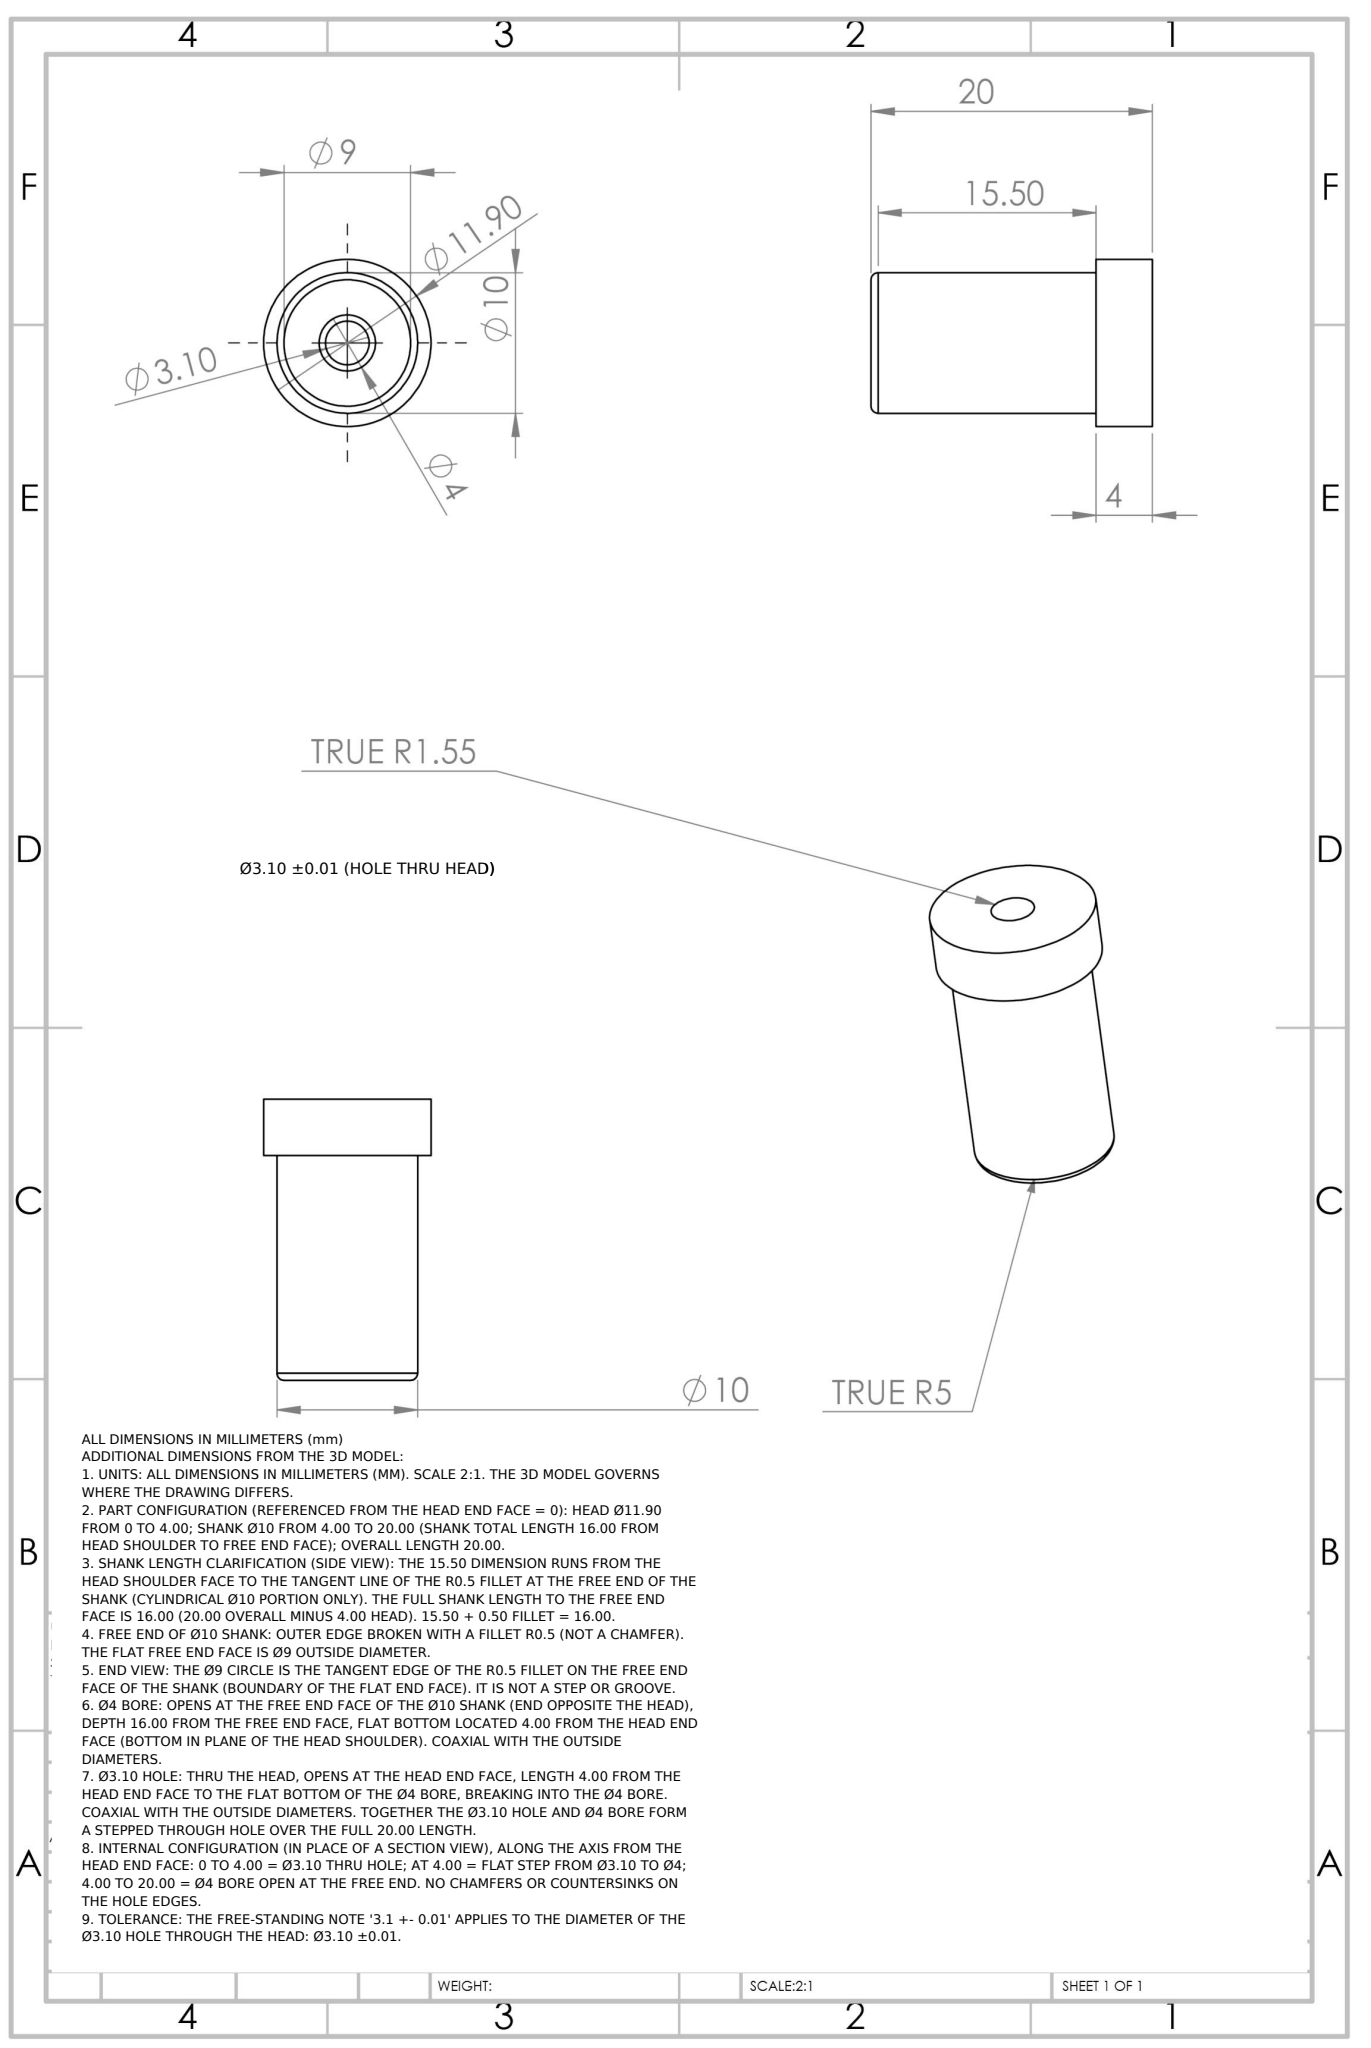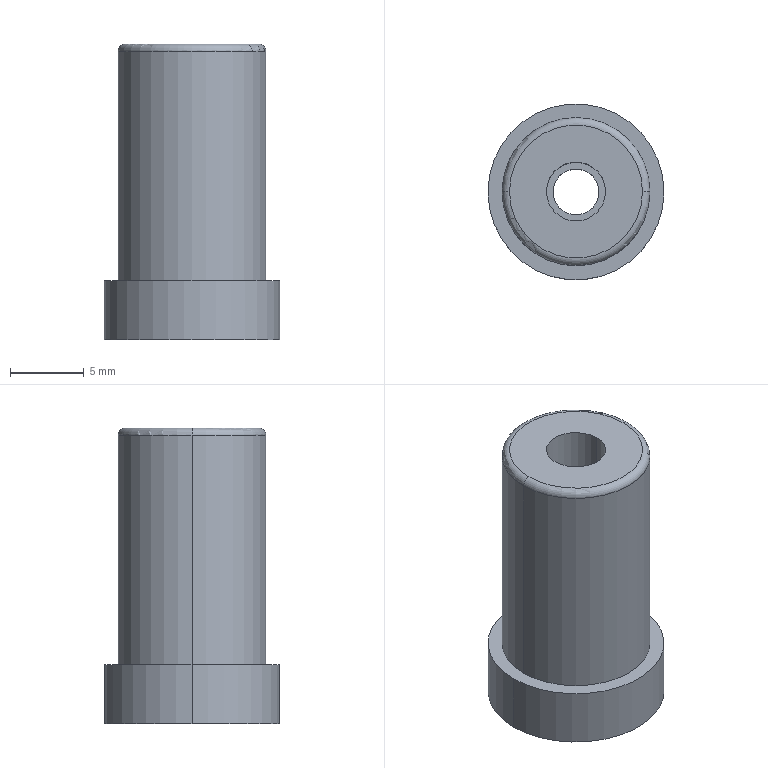Part | NX | mm | Flanged Cylindrical Bore Bushing | 1 solid | 14 faces | box 11.9 x 11.9 x 20 mm | volume 1469 mm3 | cylinder 8 | plane 4 | torus 2 | commonest cylinder face diameters 4 x2 10 x2 11.9 x2 3.1 x2
STEP:
#1=COLOUR_RGB('',1.,0.7529,1.);
#2=FILL_AREA_STYLE_COLOUR('',#1);
#3=FILL_AREA_STYLE('',(#2));
#4=SURFACE_STYLE_FILL_AREA(#3);
#5=SURFACE_SIDE_STYLE('',(#4));
#6=SURFACE_STYLE_USAGE(.BOTH.,#5);
#7=PRESENTATION_STYLE_ASSIGNMENT((#6));
#8=CARTESIAN_POINT('',(-2.,0.,4.));
#9=VERTEX_POINT('',#8);
#10=CARTESIAN_POINT('',(2.,0.,4.));
#11=VERTEX_POINT('',#10);
#12=CARTESIAN_POINT('',(0.,0.,4.));
#13=DIRECTION('',(0.,0.,1.));
#14=DIRECTION('',(1.,0.,0.));
#15=AXIS2_PLACEMENT_3D('',#12,#13,#14);
#16=CIRCLE('',#15,2.);
#17=EDGE_CURVE('',#9,#11,#16,.T.);
#18=ORIENTED_EDGE('',*,*,#17,.F.);
#19=CARTESIAN_POINT('',(-2.,0.,20.));
#20=VERTEX_POINT('',#19);
#21=CARTESIAN_POINT('',(-2.,0.,4.));
#22=DIRECTION('',(0.,0.,1.));
#23=VECTOR('',#22,1000.);
#24=LINE('',#21,#23);
#25=EDGE_CURVE('',#9,#20,#24,.T.);
#26=ORIENTED_EDGE('',*,*,#25,.T.);
#27=CARTESIAN_POINT('',(2.,0.,20.));
#28=VERTEX_POINT('',#27);
#29=CARTESIAN_POINT('',(0.,0.,20.));
#30=DIRECTION('',(0.,0.,1.));
#31=DIRECTION('',(1.,0.,0.));
#32=AXIS2_PLACEMENT_3D('',#29,#30,#31);
#33=CIRCLE('',#32,2.);
#34=EDGE_CURVE('',#20,#28,#33,.T.);
#35=ORIENTED_EDGE('',*,*,#34,.T.);
#36=CARTESIAN_POINT('',(2.,0.,4.));
#37=DIRECTION('',(0.,0.,1.));
#38=VECTOR('',#37,1000.);
#39=LINE('',#36,#38);
#40=EDGE_CURVE('',#11,#28,#39,.T.);
#41=ORIENTED_EDGE('',*,*,#40,.F.);
#42=EDGE_LOOP('',(#18,#26,#35,#41));
#43=FACE_OUTER_BOUND('',#42,.T.);
#44=CARTESIAN_POINT('',(0.,0.,4.));
#45=DIRECTION('',(0.,0.,1.));
#46=DIRECTION('',(1.,0.,0.));
#47=AXIS2_PLACEMENT_3D('',#44,#45,#46);
#48=CYLINDRICAL_SURFACE('',#47,2.);
#49=ADVANCED_FACE('',(#43),#48,.F.);
#50=CARTESIAN_POINT('',(-5.,0.,19.5));
#51=VERTEX_POINT('',#50);
#52=CARTESIAN_POINT('',(5.,0.,19.5));
#53=VERTEX_POINT('',#52);
#54=CARTESIAN_POINT('',(0.,0.,19.5));
#55=DIRECTION('',(0.,0.,-1.));
#56=DIRECTION('',(1.,0.,0.));
#57=AXIS2_PLACEMENT_3D('',#54,#55,#56);
#58=CIRCLE('',#57,5.);
#59=EDGE_CURVE('',#51,#53,#58,.T.);
#60=ORIENTED_EDGE('',*,*,#59,.F.);
#61=CARTESIAN_POINT('',(-4.5,0.,20.));
#62=VERTEX_POINT('',#61);
#63=CARTESIAN_POINT('',(-4.5,0.,19.5));
#64=DIRECTION('',(0.,1.,0.));
#65=DIRECTION('',(-1.,0.,0.));
#66=AXIS2_PLACEMENT_3D('',#63,#64,#65);
#67=CIRCLE('',#66,0.5);
#68=EDGE_CURVE('',#51,#62,#67,.T.);
#69=ORIENTED_EDGE('',*,*,#68,.T.);
#70=CARTESIAN_POINT('',(4.5,0.,20.));
#71=VERTEX_POINT('',#70);
#72=CARTESIAN_POINT('',(0.,0.,20.));
#73=DIRECTION('',(0.,0.,1.));
#74=DIRECTION('',(1.,0.,0.));
#75=AXIS2_PLACEMENT_3D('',#72,#73,#74);
#76=CIRCLE('',#75,4.5);
#77=EDGE_CURVE('',#71,#62,#76,.T.);
#78=ORIENTED_EDGE('',*,*,#77,.F.);
#79=CARTESIAN_POINT('',(4.5,0.,19.5));
#80=DIRECTION('',(0.,-1.,0.));
#81=DIRECTION('',(0.,0.,-1.));
#82=AXIS2_PLACEMENT_3D('',#79,#80,#81);
#83=CIRCLE('',#82,0.5);
#84=EDGE_CURVE('',#53,#71,#83,.T.);
#85=ORIENTED_EDGE('',*,*,#84,.F.);
#86=EDGE_LOOP('',(#60,#69,#78,#85));
#87=FACE_OUTER_BOUND('',#86,.T.);
#88=CARTESIAN_POINT('',(0.,0.,19.5));
#89=DIRECTION('',(0.,0.,1.));
#90=DIRECTION('',(1.,0.,0.));
#91=AXIS2_PLACEMENT_3D('',#88,#89,#90);
#92=TOROIDAL_SURFACE('',#91,4.5,0.5);
#93=ADVANCED_FACE('',(#87),#92,.T.);
#94=CARTESIAN_POINT('',(5.,0.,4.));
#95=VERTEX_POINT('',#94);
#96=CARTESIAN_POINT('',(-5.,0.,4.));
#97=VERTEX_POINT('',#96);
#98=CARTESIAN_POINT('',(0.,0.,4.));
#99=DIRECTION('',(0.,0.,1.));
#100=DIRECTION('',(1.,0.,0.));
#101=AXIS2_PLACEMENT_3D('',#98,#99,#100);
#102=CIRCLE('',#101,5.);
#103=EDGE_CURVE('',#95,#97,#102,.T.);
#104=ORIENTED_EDGE('',*,*,#103,.T.);
#105=CARTESIAN_POINT('',(-5.,0.,4.));
#106=DIRECTION('',(0.,0.,1.));
#107=VECTOR('',#106,1000.);
#108=LINE('',#105,#107);
#109=EDGE_CURVE('',#97,#51,#108,.T.);
#110=ORIENTED_EDGE('',*,*,#109,.T.);
#111=ORIENTED_EDGE('',*,*,#59,.T.);
#112=CARTESIAN_POINT('',(5.,0.,4.));
#113=DIRECTION('',(0.,0.,1.));
#114=VECTOR('',#113,1000.);
#115=LINE('',#112,#114);
#116=EDGE_CURVE('',#95,#53,#115,.T.);
#117=ORIENTED_EDGE('',*,*,#116,.F.);
#118=EDGE_LOOP('',(#104,#110,#111,#117));
#119=FACE_OUTER_BOUND('',#118,.T.);
#120=CARTESIAN_POINT('',(0.,0.,4.));
#121=DIRECTION('',(0.,0.,1.));
#122=DIRECTION('',(1.,0.,0.));
#123=AXIS2_PLACEMENT_3D('',#120,#121,#122);
#124=CYLINDRICAL_SURFACE('',#123,5.);
#125=ADVANCED_FACE('',(#119),#124,.T.);
#126=CARTESIAN_POINT('',(5.95,0.,4.));
#127=VERTEX_POINT('',#126);
#128=CARTESIAN_POINT('',(-5.95,0.,4.));
#129=VERTEX_POINT('',#128);
#130=CARTESIAN_POINT('',(0.,0.,4.));
#131=DIRECTION('',(0.,0.,1.));
#132=DIRECTION('',(1.,0.,0.));
#133=AXIS2_PLACEMENT_3D('',#130,#131,#132);
#134=CIRCLE('',#133,5.95);
#135=EDGE_CURVE('',#127,#129,#134,.T.);
#136=ORIENTED_EDGE('',*,*,#135,.F.);
#137=CARTESIAN_POINT('',(5.95,0.,0.));
#138=VERTEX_POINT('',#137);
#139=CARTESIAN_POINT('',(5.95,0.,20.));
#140=DIRECTION('',(0.,0.,-1.));
#141=VECTOR('',#140,1000.);
#142=LINE('',#139,#141);
#143=EDGE_CURVE('',#127,#138,#142,.T.);
#144=ORIENTED_EDGE('',*,*,#143,.T.);
#145=CARTESIAN_POINT('',(-5.95,0.,0.));
#146=VERTEX_POINT('',#145);
#147=CARTESIAN_POINT('',(0.,0.,0.));
#148=DIRECTION('',(0.,0.,1.));
#149=DIRECTION('',(1.,0.,0.));
#150=AXIS2_PLACEMENT_3D('',#147,#148,#149);
#151=CIRCLE('',#150,5.95);
#152=EDGE_CURVE('',#138,#146,#151,.T.);
#153=ORIENTED_EDGE('',*,*,#152,.T.);
#154=CARTESIAN_POINT('',(-5.95,0.,20.));
#155=DIRECTION('',(0.,0.,-1.));
#156=VECTOR('',#155,1000.);
#157=LINE('',#154,#156);
#158=EDGE_CURVE('',#129,#146,#157,.T.);
#159=ORIENTED_EDGE('',*,*,#158,.F.);
#160=EDGE_LOOP('',(#136,#144,#153,#159));
#161=FACE_OUTER_BOUND('',#160,.T.);
#162=CARTESIAN_POINT('',(0.,0.,20.));
#163=DIRECTION('',(0.,0.,-1.));
#164=DIRECTION('',(-1.,0.,0.));
#165=AXIS2_PLACEMENT_3D('',#162,#163,#164);
#166=CYLINDRICAL_SURFACE('',#165,5.95);
#167=ADVANCED_FACE('',(#161),#166,.T.);
#168=CARTESIAN_POINT('',(1.55,0.,4.));
#169=VERTEX_POINT('',#168);
#170=CARTESIAN_POINT('',(-1.55,0.,4.));
#171=VERTEX_POINT('',#170);
#172=CARTESIAN_POINT('',(0.,0.,4.));
#173=DIRECTION('',(0.,0.,-1.));
#174=DIRECTION('',(1.,0.,0.));
#175=AXIS2_PLACEMENT_3D('',#172,#173,#174);
#176=CIRCLE('',#175,1.55);
#177=EDGE_CURVE('',#169,#171,#176,.T.);
#178=ORIENTED_EDGE('',*,*,#177,.F.);
#179=CARTESIAN_POINT('',(1.55,0.,0.));
#180=VERTEX_POINT('',#179);
#181=CARTESIAN_POINT('',(1.55,0.,20.));
#182=DIRECTION('',(0.,0.,-1.));
#183=VECTOR('',#182,1000.);
#184=LINE('',#181,#183);
#185=EDGE_CURVE('',#169,#180,#184,.T.);
#186=ORIENTED_EDGE('',*,*,#185,.T.);
#187=CARTESIAN_POINT('',(-1.55,0.,0.));
#188=VERTEX_POINT('',#187);
#189=CARTESIAN_POINT('',(0.,0.,0.));
#190=DIRECTION('',(0.,0.,-1.));
#191=DIRECTION('',(-1.,0.,0.));
#192=AXIS2_PLACEMENT_3D('',#189,#190,#191);
#193=CIRCLE('',#192,1.55);
#194=EDGE_CURVE('',#180,#188,#193,.T.);
#195=ORIENTED_EDGE('',*,*,#194,.T.);
#196=CARTESIAN_POINT('',(-1.55,0.,20.));
#197=DIRECTION('',(0.,0.,-1.));
#198=VECTOR('',#197,1000.);
#199=LINE('',#196,#198);
#200=EDGE_CURVE('',#171,#188,#199,.T.);
#201=ORIENTED_EDGE('',*,*,#200,.F.);
#202=EDGE_LOOP('',(#178,#186,#195,#201));
#203=FACE_OUTER_BOUND('',#202,.T.);
#204=CARTESIAN_POINT('',(0.,0.,20.));
#205=DIRECTION('',(0.,0.,-1.));
#206=DIRECTION('',(-1.,0.,0.));
#207=AXIS2_PLACEMENT_3D('',#204,#205,#206);
#208=CYLINDRICAL_SURFACE('',#207,1.55);
#209=ADVANCED_FACE('',(#203),#208,.F.);
#210=ORIENTED_EDGE('',*,*,#185,.F.);
#211=CARTESIAN_POINT('',(0.,0.,4.));
#212=DIRECTION('',(0.,0.,-1.));
#213=DIRECTION('',(1.,0.,0.));
#214=AXIS2_PLACEMENT_3D('',#211,#212,#213);
#215=CIRCLE('',#214,1.55);
#216=EDGE_CURVE('',#171,#169,#215,.T.);
#217=ORIENTED_EDGE('',*,*,#216,.F.);
#218=ORIENTED_EDGE('',*,*,#200,.T.);
#219=CARTESIAN_POINT('',(0.,0.,0.));
#220=DIRECTION('',(0.,0.,-1.));
#221=DIRECTION('',(-1.,0.,0.));
#222=AXIS2_PLACEMENT_3D('',#219,#220,#221);
#223=CIRCLE('',#222,1.55);
#224=EDGE_CURVE('',#188,#180,#223,.T.);
#225=ORIENTED_EDGE('',*,*,#224,.T.);
#226=EDGE_LOOP('',(#210,#217,#218,#225));
#227=FACE_OUTER_BOUND('',#226,.T.);
#228=CARTESIAN_POINT('',(0.,0.,20.));
#229=DIRECTION('',(0.,0.,-1.));
#230=DIRECTION('',(-1.,0.,0.));
#231=AXIS2_PLACEMENT_3D('',#228,#229,#230);
#232=CYLINDRICAL_SURFACE('',#231,1.55);
#233=ADVANCED_FACE('',(#227),#232,.F.);
#234=ORIENTED_EDGE('',*,*,#143,.F.);
#235=CARTESIAN_POINT('',(0.,0.,4.));
#236=DIRECTION('',(0.,0.,1.));
#237=DIRECTION('',(1.,0.,0.));
#238=AXIS2_PLACEMENT_3D('',#235,#236,#237);
#239=CIRCLE('',#238,5.95);
#240=EDGE_CURVE('',#129,#127,#239,.T.);
#241=ORIENTED_EDGE('',*,*,#240,.F.);
#242=ORIENTED_EDGE('',*,*,#158,.T.);
#243=CARTESIAN_POINT('',(0.,0.,0.));
#244=DIRECTION('',(0.,0.,1.));
#245=DIRECTION('',(1.,0.,0.));
#246=AXIS2_PLACEMENT_3D('',#243,#244,#245);
#247=CIRCLE('',#246,5.95);
#248=EDGE_CURVE('',#146,#138,#247,.T.);
#249=ORIENTED_EDGE('',*,*,#248,.T.);
#250=EDGE_LOOP('',(#234,#241,#242,#249));
#251=FACE_OUTER_BOUND('',#250,.T.);
#252=CARTESIAN_POINT('',(0.,0.,20.));
#253=DIRECTION('',(0.,0.,-1.));
#254=DIRECTION('',(-1.,0.,0.));
#255=AXIS2_PLACEMENT_3D('',#252,#253,#254);
#256=CYLINDRICAL_SURFACE('',#255,5.95);
#257=ADVANCED_FACE('',(#251),#256,.T.);
#258=ORIENTED_EDGE('',*,*,#224,.F.);
#259=ORIENTED_EDGE('',*,*,#194,.F.);
#260=EDGE_LOOP('',(#258,#259));
#261=FACE_BOUND('',#260,.T.);
#262=ORIENTED_EDGE('',*,*,#248,.F.);
#263=ORIENTED_EDGE('',*,*,#152,.F.);
#264=EDGE_LOOP('',(#262,#263));
#265=FACE_OUTER_BOUND('',#264,.T.);
#266=CARTESIAN_POINT('',(0.,0.,0.));
#267=DIRECTION('',(0.,0.,1.));
#268=DIRECTION('',(1.,0.,0.));
#269=AXIS2_PLACEMENT_3D('',#266,#267,#268);
#270=PLANE('',#269);
#271=ADVANCED_FACE('',(#261,#265),#270,.F.);
#272=ORIENTED_EDGE('',*,*,#103,.F.);
#273=CARTESIAN_POINT('',(0.,0.,4.));
#274=DIRECTION('',(0.,0.,1.));
#275=DIRECTION('',(1.,0.,0.));
#276=AXIS2_PLACEMENT_3D('',#273,#274,#275);
#277=CIRCLE('',#276,5.);
#278=EDGE_CURVE('',#97,#95,#277,.T.);
#279=ORIENTED_EDGE('',*,*,#278,.F.);
#280=EDGE_LOOP('',(#272,#279));
#281=FACE_BOUND('',#280,.T.);
#282=ORIENTED_EDGE('',*,*,#240,.T.);
#283=ORIENTED_EDGE('',*,*,#135,.T.);
#284=EDGE_LOOP('',(#282,#283));
#285=FACE_OUTER_BOUND('',#284,.T.);
#286=CARTESIAN_POINT('',(0.,0.,4.));
#287=DIRECTION('',(0.,0.,1.));
#288=DIRECTION('',(1.,0.,0.));
#289=AXIS2_PLACEMENT_3D('',#286,#287,#288);
#290=PLANE('',#289);
#291=ADVANCED_FACE('',(#281,#285),#290,.T.);
#292=ORIENTED_EDGE('',*,*,#109,.F.);
#293=ORIENTED_EDGE('',*,*,#278,.T.);
#294=ORIENTED_EDGE('',*,*,#116,.T.);
#295=CARTESIAN_POINT('',(0.,0.,19.5));
#296=DIRECTION('',(0.,0.,-1.));
#297=DIRECTION('',(1.,0.,0.));
#298=AXIS2_PLACEMENT_3D('',#295,#296,#297);
#299=CIRCLE('',#298,5.);
#300=EDGE_CURVE('',#53,#51,#299,.T.);
#301=ORIENTED_EDGE('',*,*,#300,.T.);
#302=EDGE_LOOP('',(#292,#293,#294,#301));
#303=FACE_OUTER_BOUND('',#302,.T.);
#304=CARTESIAN_POINT('',(0.,0.,4.));
#305=DIRECTION('',(0.,0.,1.));
#306=DIRECTION('',(1.,0.,0.));
#307=AXIS2_PLACEMENT_3D('',#304,#305,#306);
#308=CYLINDRICAL_SURFACE('',#307,5.);
#309=ADVANCED_FACE('',(#303),#308,.T.);
#310=CARTESIAN_POINT('',(0.,0.,20.));
#311=DIRECTION('',(0.,0.,1.));
#312=DIRECTION('',(1.,0.,0.));
#313=AXIS2_PLACEMENT_3D('',#310,#311,#312);
#314=CIRCLE('',#313,2.);
#315=EDGE_CURVE('',#28,#20,#314,.T.);
#316=ORIENTED_EDGE('',*,*,#315,.F.);
#317=ORIENTED_EDGE('',*,*,#34,.F.);
#318=EDGE_LOOP('',(#316,#317));
#319=FACE_BOUND('',#318,.T.);
#320=ORIENTED_EDGE('',*,*,#77,.T.);
#321=CARTESIAN_POINT('',(0.,0.,20.));
#322=DIRECTION('',(0.,0.,1.));
#323=DIRECTION('',(1.,0.,0.));
#324=AXIS2_PLACEMENT_3D('',#321,#322,#323);
#325=CIRCLE('',#324,4.5);
#326=EDGE_CURVE('',#62,#71,#325,.T.);
#327=ORIENTED_EDGE('',*,*,#326,.T.);
#328=EDGE_LOOP('',(#320,#327));
#329=FACE_OUTER_BOUND('',#328,.T.);
#330=CARTESIAN_POINT('',(0.,0.,20.));
#331=DIRECTION('',(0.,0.,1.));
#332=DIRECTION('',(1.,0.,0.));
#333=AXIS2_PLACEMENT_3D('',#330,#331,#332);
#334=PLANE('',#333);
#335=ADVANCED_FACE('',(#319,#329),#334,.T.);
#336=ORIENTED_EDGE('',*,*,#68,.F.);
#337=ORIENTED_EDGE('',*,*,#300,.F.);
#338=ORIENTED_EDGE('',*,*,#84,.T.);
#339=ORIENTED_EDGE('',*,*,#326,.F.);
#340=EDGE_LOOP('',(#336,#337,#338,#339));
#341=FACE_OUTER_BOUND('',#340,.T.);
#342=CARTESIAN_POINT('',(0.,0.,19.5));
#343=DIRECTION('',(0.,0.,1.));
#344=DIRECTION('',(1.,0.,0.));
#345=AXIS2_PLACEMENT_3D('',#342,#343,#344);
#346=TOROIDAL_SURFACE('',#345,4.5,0.5);
#347=ADVANCED_FACE('',(#341),#346,.T.);
#348=CARTESIAN_POINT('',(0.,0.,4.));
#349=DIRECTION('',(0.,0.,1.));
#350=DIRECTION('',(1.,0.,0.));
#351=AXIS2_PLACEMENT_3D('',#348,#349,#350);
#352=CIRCLE('',#351,2.);
#353=EDGE_CURVE('',#11,#9,#352,.T.);
#354=ORIENTED_EDGE('',*,*,#353,.T.);
#355=ORIENTED_EDGE('',*,*,#17,.T.);
#356=EDGE_LOOP('',(#354,#355));
#357=FACE_OUTER_BOUND('',#356,.T.);
#358=ORIENTED_EDGE('',*,*,#216,.T.);
#359=ORIENTED_EDGE('',*,*,#177,.T.);
#360=EDGE_LOOP('',(#358,#359));
#361=FACE_BOUND('',#360,.T.);
#362=CARTESIAN_POINT('',(0.,0.,4.));
#363=DIRECTION('',(0.,0.,1.));
#364=DIRECTION('',(1.,0.,0.));
#365=AXIS2_PLACEMENT_3D('',#362,#363,#364);
#366=PLANE('',#365);
#367=ADVANCED_FACE('',(#357,#361),#366,.T.);
#368=ORIENTED_EDGE('',*,*,#25,.F.);
#369=ORIENTED_EDGE('',*,*,#353,.F.);
#370=ORIENTED_EDGE('',*,*,#40,.T.);
#371=ORIENTED_EDGE('',*,*,#315,.T.);
#372=EDGE_LOOP('',(#368,#369,#370,#371));
#373=FACE_OUTER_BOUND('',#372,.T.);
#374=CARTESIAN_POINT('',(0.,0.,4.));
#375=DIRECTION('',(0.,0.,1.));
#376=DIRECTION('',(1.,0.,0.));
#377=AXIS2_PLACEMENT_3D('',#374,#375,#376);
#378=CYLINDRICAL_SURFACE('',#377,2.);
#379=ADVANCED_FACE('',(#373),#378,.F.);
#380=CLOSED_SHELL('',(#49,#93,#125,#167,#209,#233,#257,#271,#291,#309,#335,#347,#367,#379));
#381=MANIFOLD_SOLID_BREP('',#380);
#382=STYLED_ITEM('',(#7),#381);
#383=(LENGTH_UNIT()NAMED_UNIT(*)SI_UNIT(.MILLI.,.METRE.));
#384=UNCERTAINTY_MEASURE_WITH_UNIT(LENGTH_MEASURE(0.00001),#383,'','');
#385=(NAMED_UNIT(*)PLANE_ANGLE_UNIT()SI_UNIT($,.RADIAN.));
#386=(NAMED_UNIT(*)SI_UNIT($,.STERADIAN.)SOLID_ANGLE_UNIT());
#387=(GEOMETRIC_REPRESENTATION_CONTEXT(3)GLOBAL_UNCERTAINTY_ASSIGNED_CONTEXT((#384))GLOBAL_UNIT_ASSIGNED_CONTEXT((#383,#385,#386))REPRESENTATION_CONTEXT('',''));
#388=MECHANICAL_DESIGN_GEOMETRIC_PRESENTATION_REPRESENTATION('',(#382),#387);
#389=PRESENTATION_LAYER_ASSIGNMENT('','',(#382));
#390=COLOUR_RGB('',0.7922,0.8196,0.9333);
#391=FILL_AREA_STYLE_COLOUR('',#390);
#392=FILL_AREA_STYLE('',(#391));
#393=SURFACE_STYLE_FILL_AREA(#392);
#394=SURFACE_SIDE_STYLE('',(#393));
#395=SURFACE_STYLE_USAGE(.BOTH.,#394);
#396=PRESENTATION_STYLE_ASSIGNMENT((#395));
#397=CARTESIAN_POINT('',(0.,0.,0.));
#398=DIRECTION('',(0.,0.,1.));
#399=DIRECTION('',(1.,0.,0.));
#400=AXIS2_PLACEMENT_3D('',#397,#398,#399);
#401=(LENGTH_UNIT()NAMED_UNIT(*)SI_UNIT(.MILLI.,.METRE.));
#402=UNCERTAINTY_MEASURE_WITH_UNIT(LENGTH_MEASURE(0.00001),#401,'','');
#403=(NAMED_UNIT(*)PLANE_ANGLE_UNIT()SI_UNIT($,.RADIAN.));
#404=(NAMED_UNIT(*)SI_UNIT($,.STERADIAN.)SOLID_ANGLE_UNIT());
#405=(GEOMETRIC_REPRESENTATION_CONTEXT(3)GLOBAL_UNCERTAINTY_ASSIGNED_CONTEXT((#402))GLOBAL_UNIT_ASSIGNED_CONTEXT((#401,#403,#404))REPRESENTATION_CONTEXT('',''));
#406=ADVANCED_BREP_SHAPE_REPRESENTATION('',(#381,#400),#405);
#407=STYLED_ITEM('',(#396),#406);
#408=PRESENTATION_LAYER_ASSIGNMENT('','',(#407));
#409=(LENGTH_UNIT()NAMED_UNIT(*)SI_UNIT(.MILLI.,.METRE.));
#410=UNCERTAINTY_MEASURE_WITH_UNIT(LENGTH_MEASURE(0.00001),#409,'','');
#411=(NAMED_UNIT(*)PLANE_ANGLE_UNIT()SI_UNIT($,.RADIAN.));
#412=(NAMED_UNIT(*)SI_UNIT($,.STERADIAN.)SOLID_ANGLE_UNIT());
#413=(GEOMETRIC_REPRESENTATION_CONTEXT(3)GLOBAL_UNCERTAINTY_ASSIGNED_CONTEXT((#410))GLOBAL_UNIT_ASSIGNED_CONTEXT((#409,#411,#412))REPRESENTATION_CONTEXT('',''));
#414=MECHANICAL_DESIGN_GEOMETRIC_PRESENTATION_REPRESENTATION('',(#407),#413);